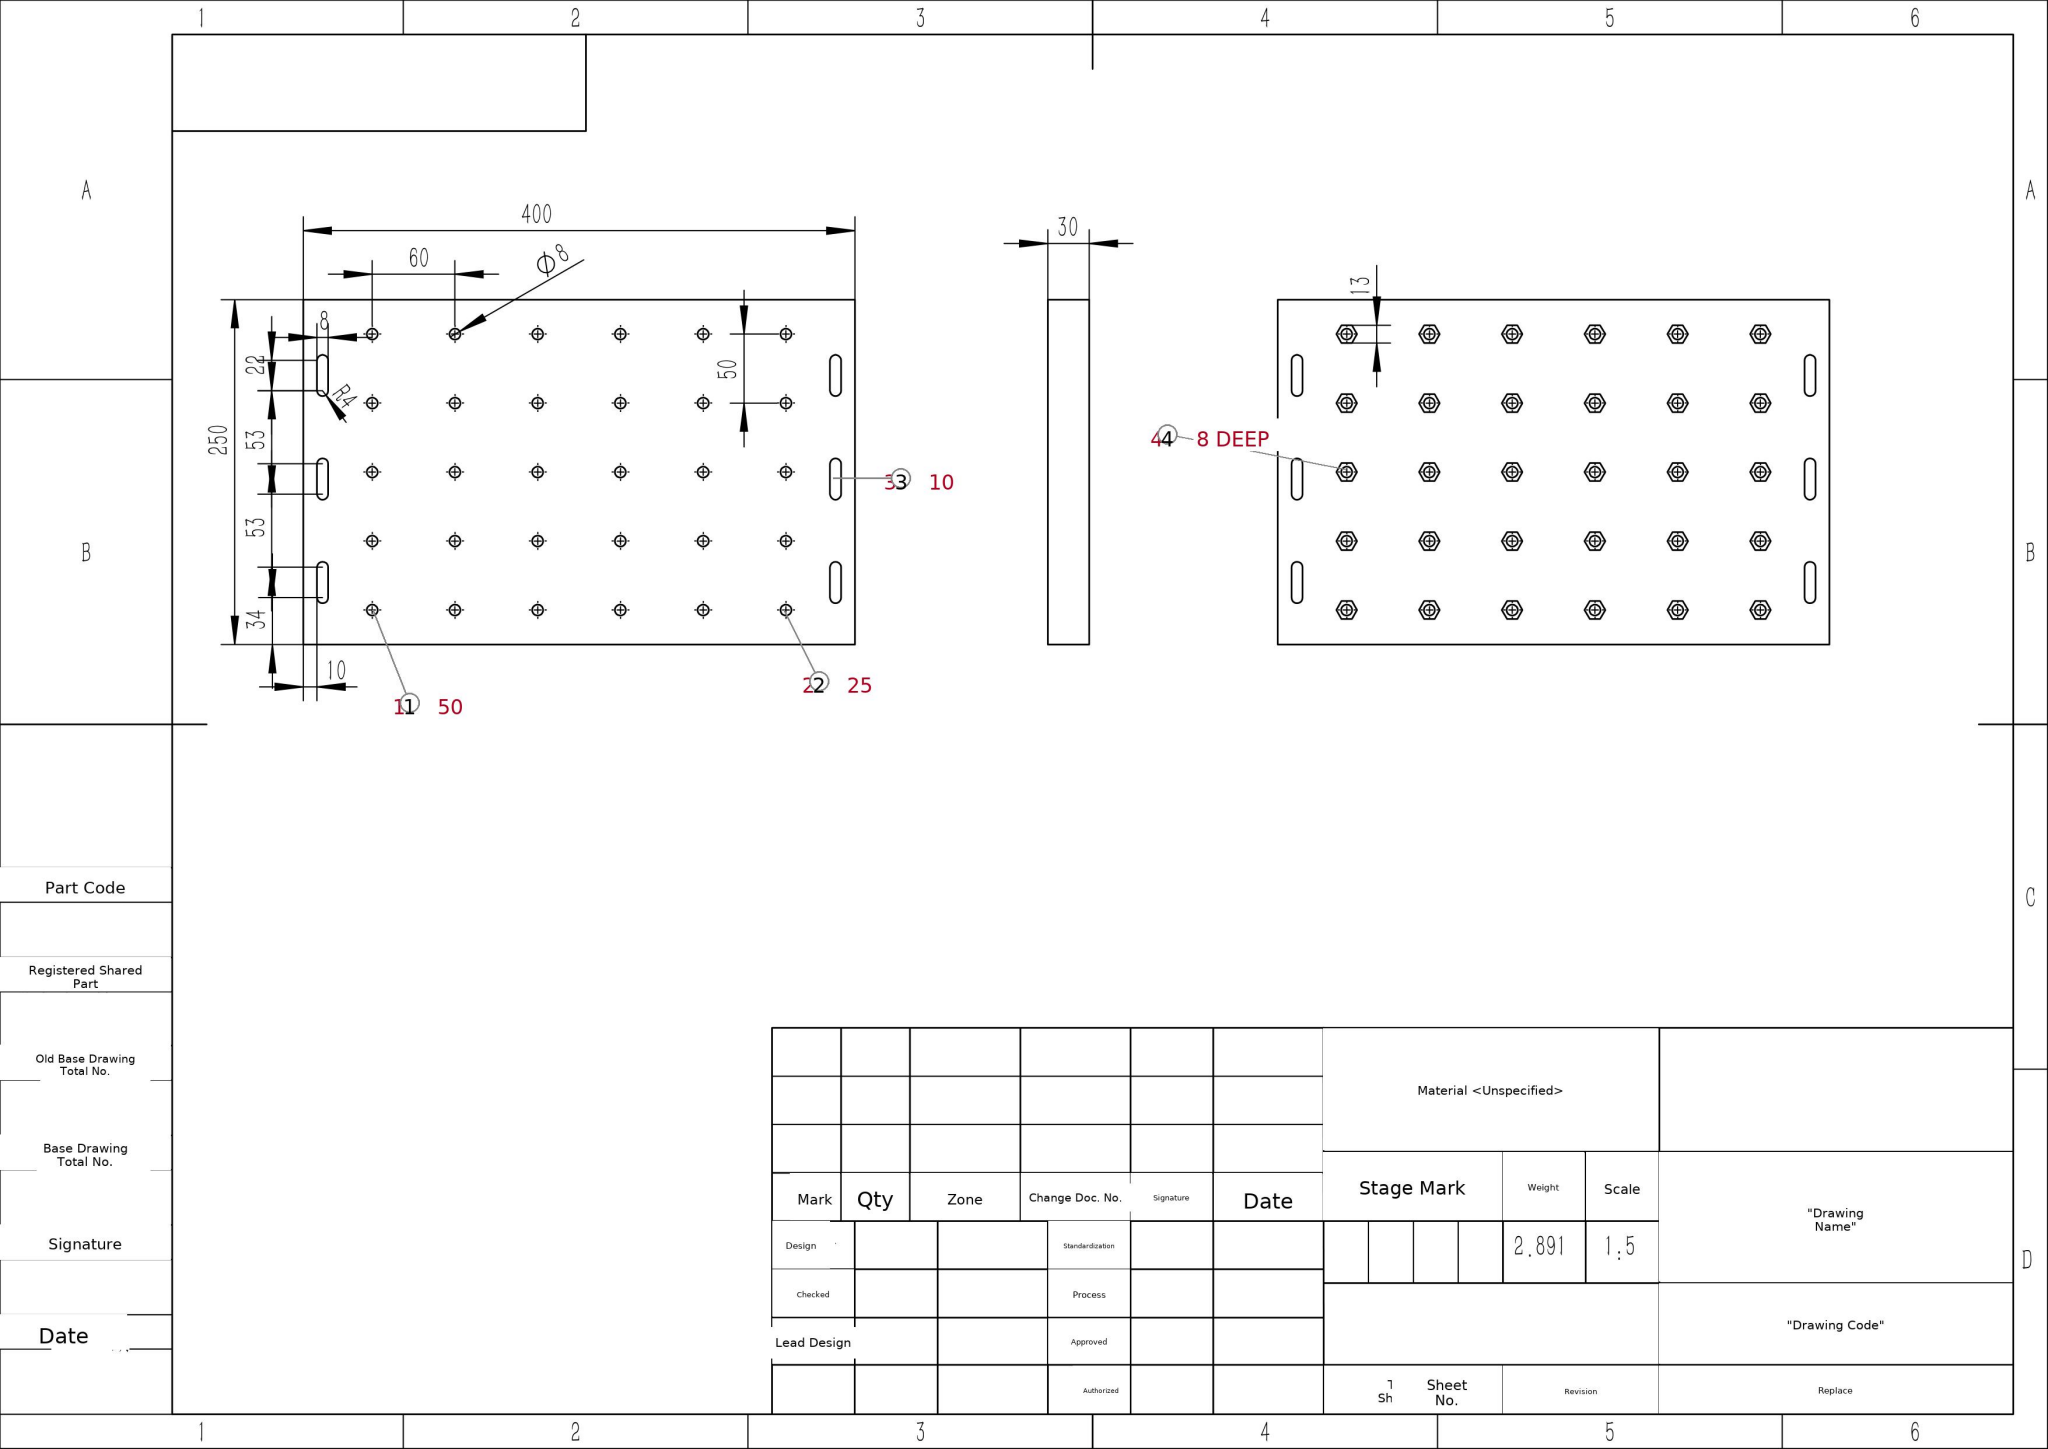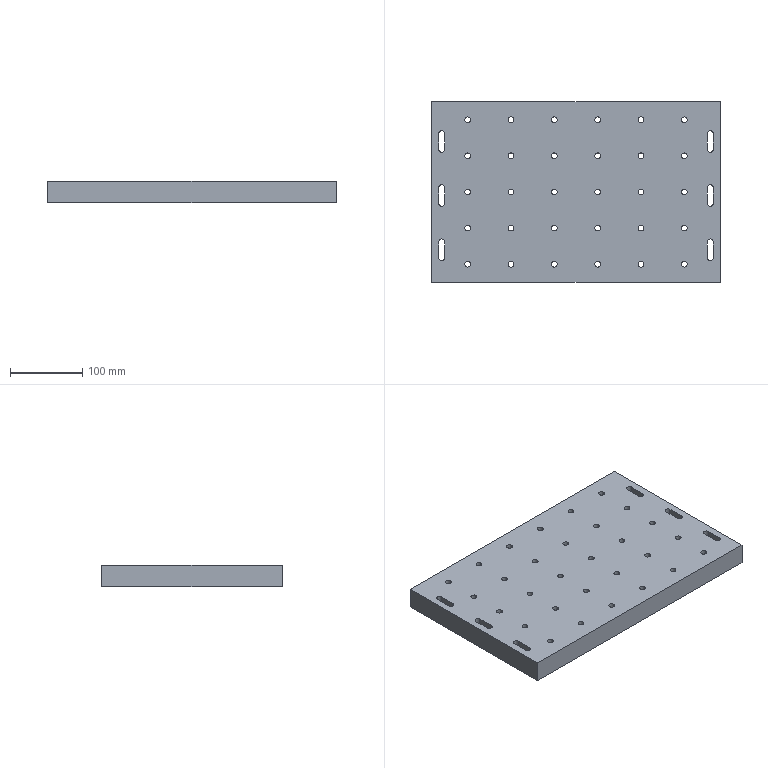Part | SolidWorks | mm | 1 solid | 300 faces | box 400 x 250 x 30 mm | volume 2890971 mm3 | plane 228 | cylinder 72 | commonest cylinder face diameters 8 x72
build123d program:
from build123d import *

# Parameters (mm, degrees)
SKETCH1_W           = 400
SKETCH1_H           = 250
BOSS_EXTRUDE1_DEPTH = 30
SKETCH2_R           = 4
CUT_EXTRUDE1_DEPTH  = 30
CUT_EXTRUDE2_DEPTH  = 8


with BuildPart() as part:
    # Sketch1 → Boss-Extrude1 (new body)
    with BuildSketch(Plane.XY):
        Rectangle(SKETCH1_W, SKETCH1_H)
    extrude(amount=BOSS_EXTRUDE1_DEPTH)

    # Sketch2 → Cut-Extrude1 (cut)
    with BuildSketch(Plane.XY.offset(30)):
        with Locations((-150, 100)):
            Circle(SKETCH2_R)
        with Locations((-90, 100)):
            Circle(SKETCH2_R)
        with Locations((-30, 100)):
            Circle(SKETCH2_R)
        with Locations((30, 100)):
            Circle(SKETCH2_R)
        with Locations((90, 100)):
            Circle(SKETCH2_R)
        with Locations((150, 100)):
            Circle(SKETCH2_R)
        with Locations((-150, 50)):
            Circle(SKETCH2_R)
        with Locations((-90, 50)):
            Circle(SKETCH2_R)
        with Locations((-30, 50)):
            Circle(SKETCH2_R)
        with Locations((30, 50)):
            Circle(SKETCH2_R)
        with Locations((90, 50)):
            Circle(SKETCH2_R)
        with Locations((150, 50)):
            Circle(SKETCH2_R)
        with Locations((-150, 0)):
            Circle(SKETCH2_R)
        with Locations((-90, 0)):
            Circle(SKETCH2_R)
        with Locations((-30, 0)):
            Circle(SKETCH2_R)
        with Locations((30, 0)):
            Circle(SKETCH2_R)
        with Locations((90, 0)):
            Circle(SKETCH2_R)
        with Locations((150, 0)):
            Circle(SKETCH2_R)
        with Locations((-150, -50)):
            Circle(SKETCH2_R)
        with Locations((-90, -50)):
            Circle(SKETCH2_R)
        with Locations((-30, -50)):
            Circle(SKETCH2_R)
        with Locations((30, -50)):
            Circle(SKETCH2_R)
        with Locations((90, -50)):
            Circle(SKETCH2_R)
        with Locations((150, -50)):
            Circle(SKETCH2_R)
        with Locations((-150, -100)):
            Circle(SKETCH2_R)
        with Locations((-90, -100)):
            Circle(SKETCH2_R)
        with Locations((-30, -100)):
            Circle(SKETCH2_R)
        with Locations((30, -100)):
            Circle(SKETCH2_R)
        with Locations((90, -100)):
            Circle(SKETCH2_R)
        with Locations((150, -100)):
            Circle(SKETCH2_R)
        with BuildLine():
            Line((-182, 81), (-182, 59))
            ThreePointArc((-182, 59), (-186, 55), (-190, 59))
            Line((-190, 59), (-190, 81))
            ThreePointArc((-190, 81), (-186, 85), (-182, 81))
        make_face()
        with BuildLine():
            Line((-182, 6), (-182, -16))
            ThreePointArc((-182, -16), (-186, -20), (-190, -16))
            Line((-190, -16), (-190, 6))
            ThreePointArc((-190, 6), (-186, 10), (-182, 6))
        make_face()
        with BuildLine():
            Line((-182, -69), (-182, -91))
            ThreePointArc((-182, -91), (-186, -95), (-190, -91))
            Line((-190, -91), (-190, -69))
            ThreePointArc((-190, -69), (-186, -65), (-182, -69))
        make_face()
        with BuildLine():
            Line((182, -69), (182, -91))
            ThreePointArc((182, -91), (186, -95), (190, -91))
            Line((190, -91), (190, -69))
            ThreePointArc((190, -69), (186, -65), (182, -69))
        make_face()
        with BuildLine():
            Line((182, 6), (182, -16))
            ThreePointArc((182, -16), (186, -20), (190, -16))
            Line((190, -16), (190, 6))
            ThreePointArc((190, 6), (186, 10), (182, 6))
        make_face()
        with BuildLine():
            Line((182, 81), (182, 59))
            ThreePointArc((182, 59), (186, 55), (190, 59))
            Line((190, 59), (190, 81))
            ThreePointArc((190, 81), (186, 85), (182, 81))
        make_face()
    extrude(amount=-CUT_EXTRUDE1_DEPTH, mode=Mode.SUBTRACT)

    # Sketch3 → Cut-Extrude2 (cut)
    with BuildSketch(Plane(origin=(0, 0, 0), x_dir=(-1, 0, 0), z_dir=(0, 0, -1))):
        Polygon((-86.247, 93.5), (-82.494, 100), (-86.247, 106.5), (-93.753, 106.5), (-97.506, 100), (-93.753, 93.5), align=None)
        Polygon((-142.494, 100), (-146.247, 106.5), (-153.753, 106.5), (-157.506, 100), (-153.753, 93.5), (-146.247, 93.5), align=None)
        Polygon((-26.247, 93.5), (-22.494, 100), (-26.247, 106.5), (-33.753, 106.5), (-37.506, 100), (-33.753, 93.5), align=None)
        Polygon((33.753, 93.5), (37.506, 100), (33.753, 106.5), (26.247, 106.5), (22.494, 100), (26.247, 93.5), align=None)
        Polygon((93.753, 93.5), (97.506, 100), (93.753, 106.5), (86.247, 106.5), (82.494, 100), (86.247, 93.5), align=None)
        Polygon((153.753, 93.5), (157.506, 100), (153.753, 106.5), (146.247, 106.5), (142.494, 100), (146.247, 93.5), align=None)
        Polygon((213.753, 93.5), (217.506, 100), (213.753, 106.5), (206.247, 106.5), (202.494, 100), (206.247, 93.5), align=None)
        Polygon((-86.247, 43.5), (-82.494, 50), (-86.247, 56.5), (-93.753, 56.5), (-97.506, 50), (-93.753, 43.5), align=None)
        Polygon((-26.247, 43.5), (-22.494, 50), (-26.247, 56.5), (-33.753, 56.5), (-37.506, 50), (-33.753, 43.5), align=None)
        Polygon((33.753, 43.5), (37.506, 50), (33.753, 56.5), (26.247, 56.5), (22.494, 50), (26.247, 43.5), align=None)
        Polygon((93.753, 43.5), (97.506, 50), (93.753, 56.5), (86.247, 56.5), (82.494, 50), (86.247, 43.5), align=None)
        Polygon((153.753, 43.5), (157.506, 50), (153.753, 56.5), (146.247, 56.5), (142.494, 50), (146.247, 43.5), align=None)
        Polygon((213.753, 43.5), (217.506, 50), (213.753, 56.5), (206.247, 56.5), (202.494, 50), (206.247, 43.5), align=None)
        Polygon((-86.247, -6.5), (-82.494, 0), (-86.247, 6.5), (-93.753, 6.5), (-97.506, 0), (-93.753, -6.5), align=None)
        Polygon((-26.247, -6.5), (-22.494, 0), (-26.247, 6.5), (-33.753, 6.5), (-37.506, 0), (-33.753, -6.5), align=None)
        Polygon((33.753, -6.5), (37.506, 0), (33.753, 6.5), (26.247, 6.5), (22.494, 0), (26.247, -6.5), align=None)
        Polygon((93.753, -6.5), (97.506, 0), (93.753, 6.5), (86.247, 6.5), (82.494, 0), (86.247, -6.5), align=None)
        Polygon((153.753, -6.5), (157.506, 0), (153.753, 6.5), (146.247, 6.5), (142.494, 0), (146.247, -6.5), align=None)
        Polygon((213.753, -6.5), (217.506, 0), (213.753, 6.5), (206.247, 6.5), (202.494, 0), (206.247, -6.5), align=None)
        Polygon((-86.247, -56.5), (-82.494, -50), (-86.247, -43.5), (-93.753, -43.5), (-97.506, -50), (-93.753, -56.5), align=None)
        Polygon((-26.247, -56.5), (-22.494, -50), (-26.247, -43.5), (-33.753, -43.5), (-37.506, -50), (-33.753, -56.5), align=None)
        Polygon((33.753, -56.5), (37.506, -50), (33.753, -43.5), (26.247, -43.5), (22.494, -50), (26.247, -56.5), align=None)
        Polygon((93.753, -56.5), (97.506, -50), (93.753, -43.5), (86.247, -43.5), (82.494, -50), (86.247, -56.5), align=None)
        Polygon((153.753, -56.5), (157.506, -50), (153.753, -43.5), (146.247, -43.5), (142.494, -50), (146.247, -56.5), align=None)
        Polygon((213.753, -56.5), (217.506, -50), (213.753, -43.5), (206.247, -43.5), (202.494, -50), (206.247, -56.5), align=None)
        Polygon((-86.247, -106.5), (-82.494, -100), (-86.247, -93.5), (-93.753, -93.5), (-97.506, -100), (-93.753, -106.5), align=None)
        Polygon((-26.247, -106.5), (-22.494, -100), (-26.247, -93.5), (-33.753, -93.5), (-37.506, -100), (-33.753, -106.5), align=None)
        Polygon((33.753, -106.5), (37.506, -100), (33.753, -93.5), (26.247, -93.5), (22.494, -100), (26.247, -106.5), align=None)
        Polygon((93.753, -106.5), (97.506, -100), (93.753, -93.5), (86.247, -93.5), (82.494, -100), (86.247, -106.5), align=None)
        Polygon((153.753, -106.5), (157.506, -100), (153.753, -93.5), (146.247, -93.5), (142.494, -100), (146.247, -106.5), align=None)
        Polygon((213.753, -106.5), (217.506, -100), (213.753, -93.5), (206.247, -93.5), (202.494, -100), (206.247, -106.5), align=None)
        Polygon((-146.247, 43.5), (-142.494, 50), (-146.247, 56.5), (-153.753, 56.5), (-157.506, 50), (-153.753, 43.5), align=None)
        Polygon((-146.247, -6.5), (-142.494, 0), (-146.247, 6.5), (-153.753, 6.5), (-157.506, 0), (-153.753, -6.5), align=None)
        Polygon((-146.247, -56.5), (-142.494, -50), (-146.247, -43.5), (-153.753, -43.5), (-157.506, -50), (-153.753, -56.5), align=None)
        Polygon((-146.247, -106.5), (-142.494, -100), (-146.247, -93.5), (-153.753, -93.5), (-157.506, -100), (-153.753, -106.5), align=None)
    extrude(amount=-CUT_EXTRUDE2_DEPTH, mode=Mode.SUBTRACT)


solid = part.part